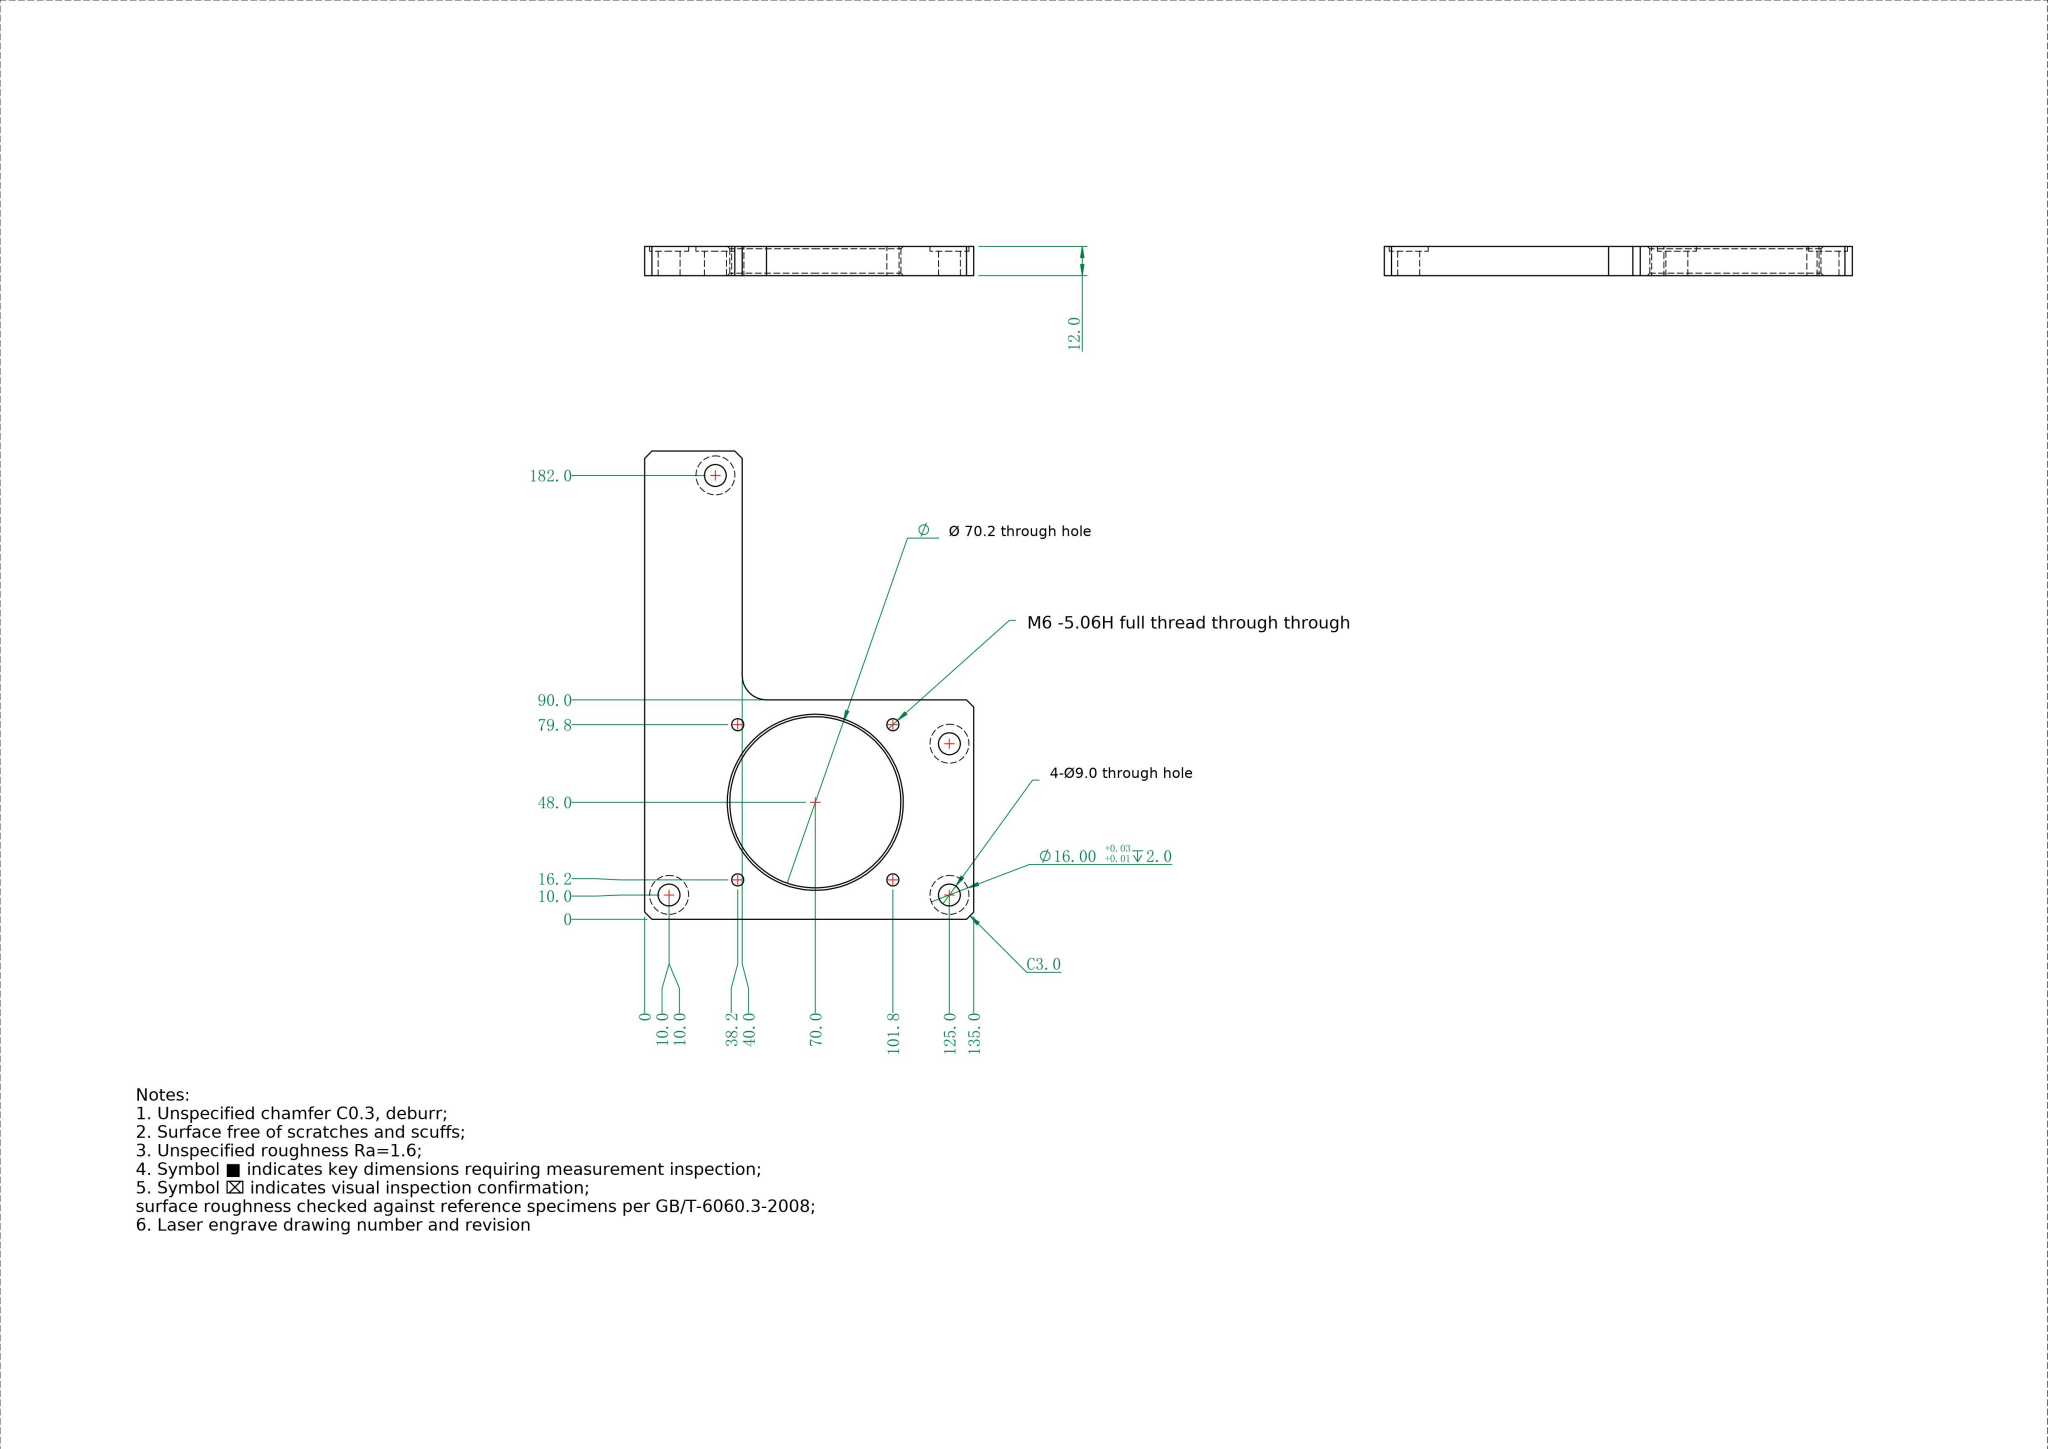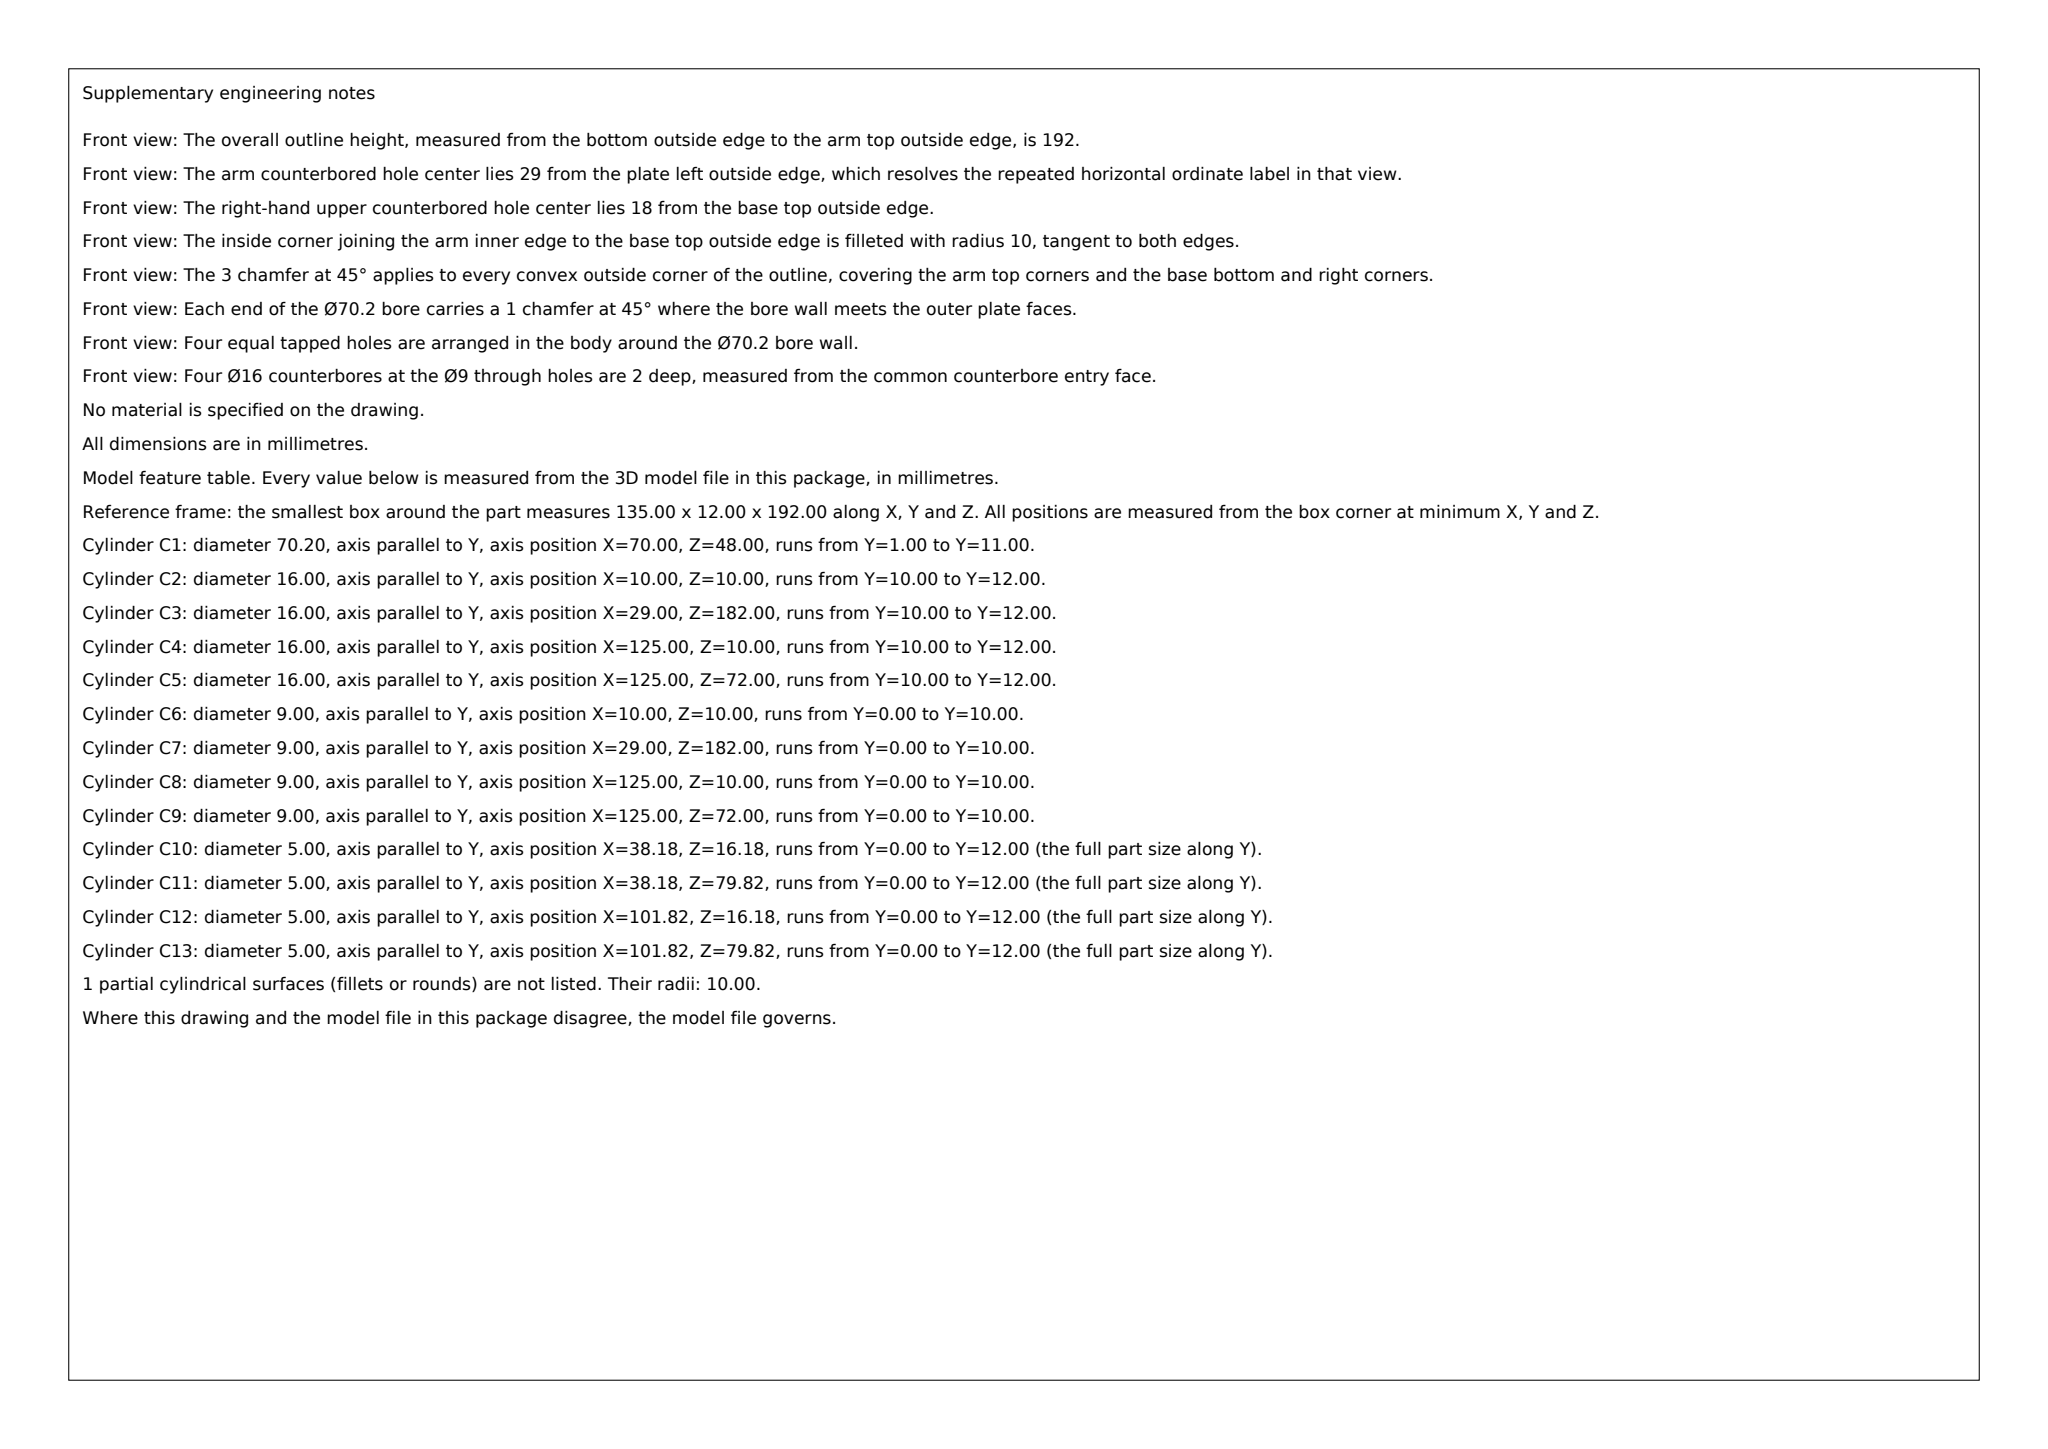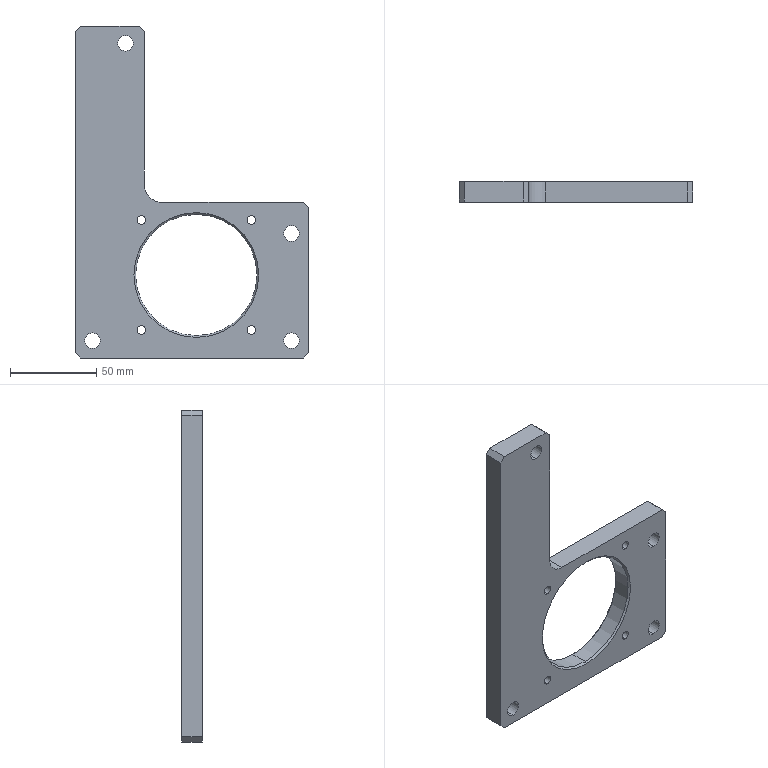Part | SolidWorks | mm | material A6061/Natural Anodized | 1 solid | 48 faces | box 135 x 12 x 192 mm | volume 142984 mm3 | cylinder 27 | plane 17 | cone 4 | commonest cylinder face diameters 16 x8 9 x8 5 x8 70.2 x2 20 x1
Drawing notes:
4X M6-5.06H FULL THREAD THRU AT X38.18/101.82, Z16.18/79.82 | from the solid: Four Ø5.0 y-axis cylinders L=12.0 (full thk) at (38.18,16.18),(38.18,79.82),(101.82,16.18),(101.82,79.82)
4X Ø9.0 THRU, Ø16.00 +0.03/+0.01 CBORE DP 2.0 | from the solid: Four Ø16.0 y-axis cylinders L=2.0 coaxial with four Ø9.0 holes at (10,10),(29,182),(125,10),(125,72)
Ø20.0 THRU AT X50.0, Z100.0 | from the solid: Ø20.0 y-axis cylinder, L=12.0 (full thk) at (50.0,100.0)
build123d program:
from build123d import *

# Parameters (mm, degrees)
SKETCH1_W                                 = 135
SKETCH1_H                                 = 192
BOSS_EXTRUDE1_DEPTH                       = 12
SKETCH2_W                                 = 95
SKETCH2_H                                 = 102
CUT_EXTRUDE1_DEPTH                        = 164.257
M6_TAPPED_HOLE1_D                         = 5
M72_CLEARANCE_HOLE2_D                     = 70.2
M8_HEX_HEAD_BOLT_COUNTERBORE1_D           = 9
M8_HEX_HEAD_BOLT_COUNTERBORE1_CBORE_D     = 16
M8_HEX_HEAD_BOLT_COUNTERBORE1_CBORE_DEPTH = 2
CHAMFER1_SIZE                             = 3
CHAMFER2_SIZE                             = 1
FILLET1_R                                 = 10


with BuildPart() as part:
    # Sketch1 → Boss-Extrude1 (new body)
    with BuildSketch(Plane(origin=(0, 6, 0), x_dir=(1, 0, 0), z_dir=(0, 1, 0))):
        with Locations((-2.5, -51)):
            Rectangle(SKETCH1_W, SKETCH1_H)
    extrude(amount=-BOSS_EXTRUDE1_DEPTH)

    # Sketch2 → Cut-Extrude1 (cut, through all)
    with BuildSketch(Plane.XZ.offset(6)):
        with Locations((17.5, 96)):
            Rectangle(SKETCH2_W, SKETCH2_H)
    extrude(amount=-CUT_EXTRUDE1_DEPTH, mode=Mode.SUBTRACT)

    # M6 Tapped Hole1 (through all)
    with Locations(Plane(origin=(0, 6, 0), x_dir=(1, 0, 0), z_dir=(0, 1, 0))):
        with Locations((-31.82, 28.82), (31.82, -34.82), (31.82, 28.82), (-31.82, -34.82)):
            Hole(M6_TAPPED_HOLE1_D / 2)

    # M72 Clearance Hole2 (through all)
    with Locations(Plane(origin=(0, 6, 0), x_dir=(1, 0, 0), z_dir=(0, 1, 0))):
        with Locations((0, -3)):
            Hole(M72_CLEARANCE_HOLE2_D / 2)

    # M8 Hex Head Bolt Counterbore1 (through all)
    with Locations(Plane(origin=(0, 6, 0), x_dir=(1, 0, 0), z_dir=(0, 1, 0))):
        with Locations((-60, 35), (55, 35), (55, -27), (-41, -137)):
            CounterBoreHole(M8_HEX_HEAD_BOLT_COUNTERBORE1_D / 2, M8_HEX_HEAD_BOLT_COUNTERBORE1_CBORE_D / 2, M8_HEX_HEAD_BOLT_COUNTERBORE1_CBORE_DEPTH)

    # Chamfer1
    chamfer1_edges = [part.edges().sort_by_distance(p)[0] for p in [
        (65, 0, 45),
        (-30, 0, 147),
        (-70, 0, -45),
        (65, 0, -45),
        (-70, 0, 147),
    ]]
    chamfer(chamfer1_edges, length=CHAMFER1_SIZE)

    # Chamfer2
    chamfer2_edges = [part.edges().sort_by_distance(p)[0] for p in [
        (35.1, 6, 3),
        (35.1, -6, 3),
    ]]
    chamfer(chamfer2_edges, length=CHAMFER2_SIZE)

    # Fillet1
    fillet1_edges = [part.edges().sort_by_distance(p)[0] for p in [
        (-30, 0, 45),
    ]]
    fillet(fillet1_edges, radius=FILLET1_R)


solid = part.part